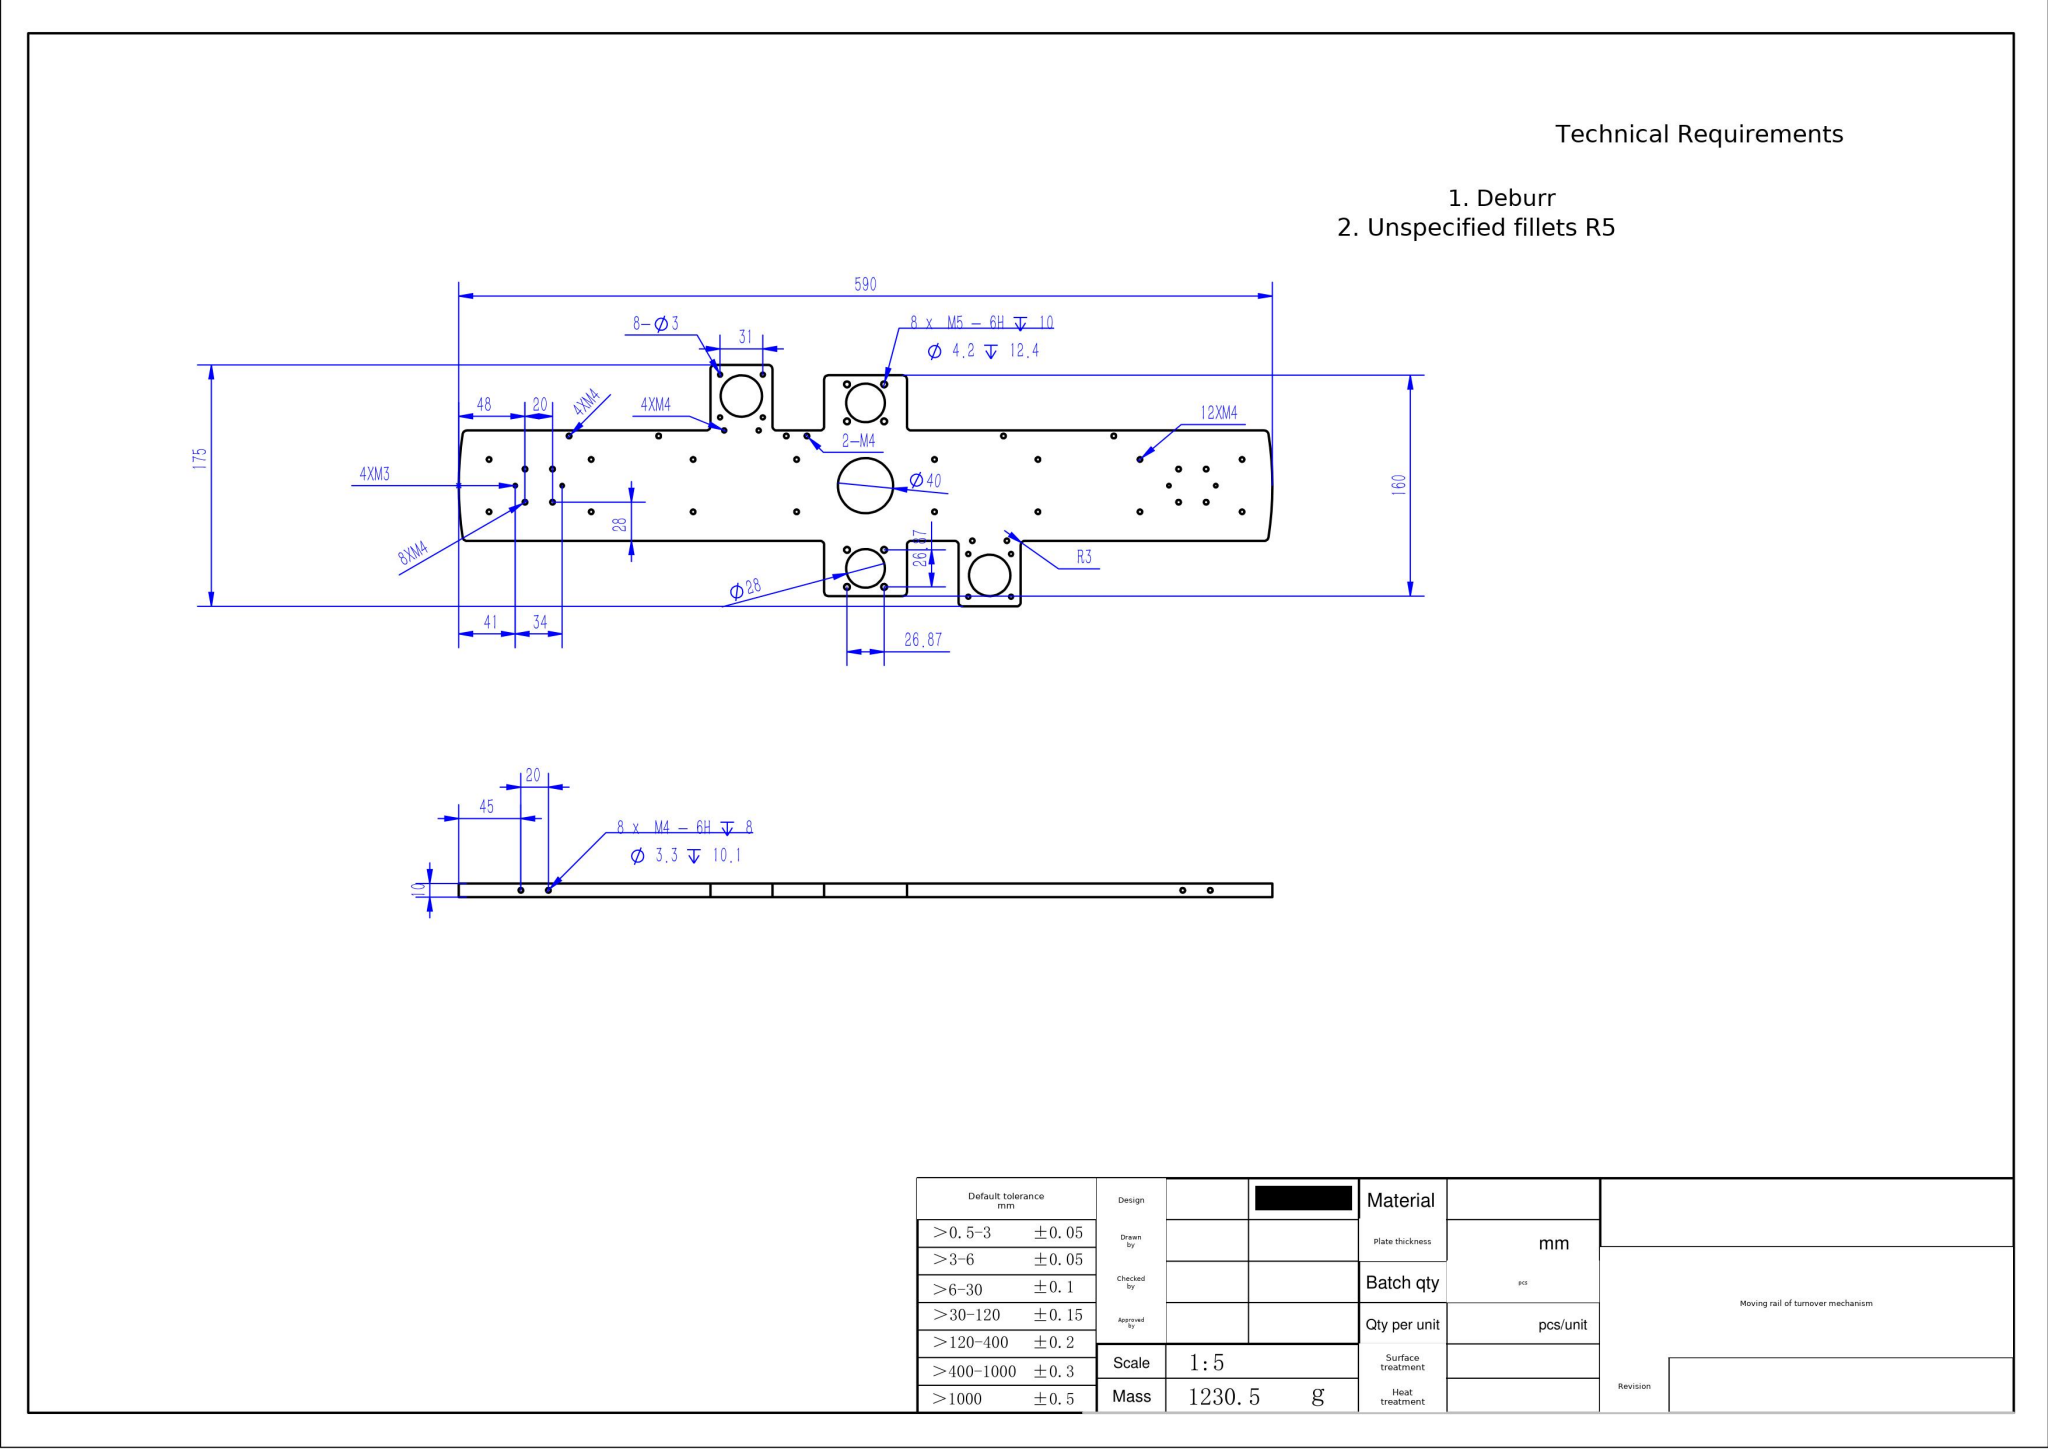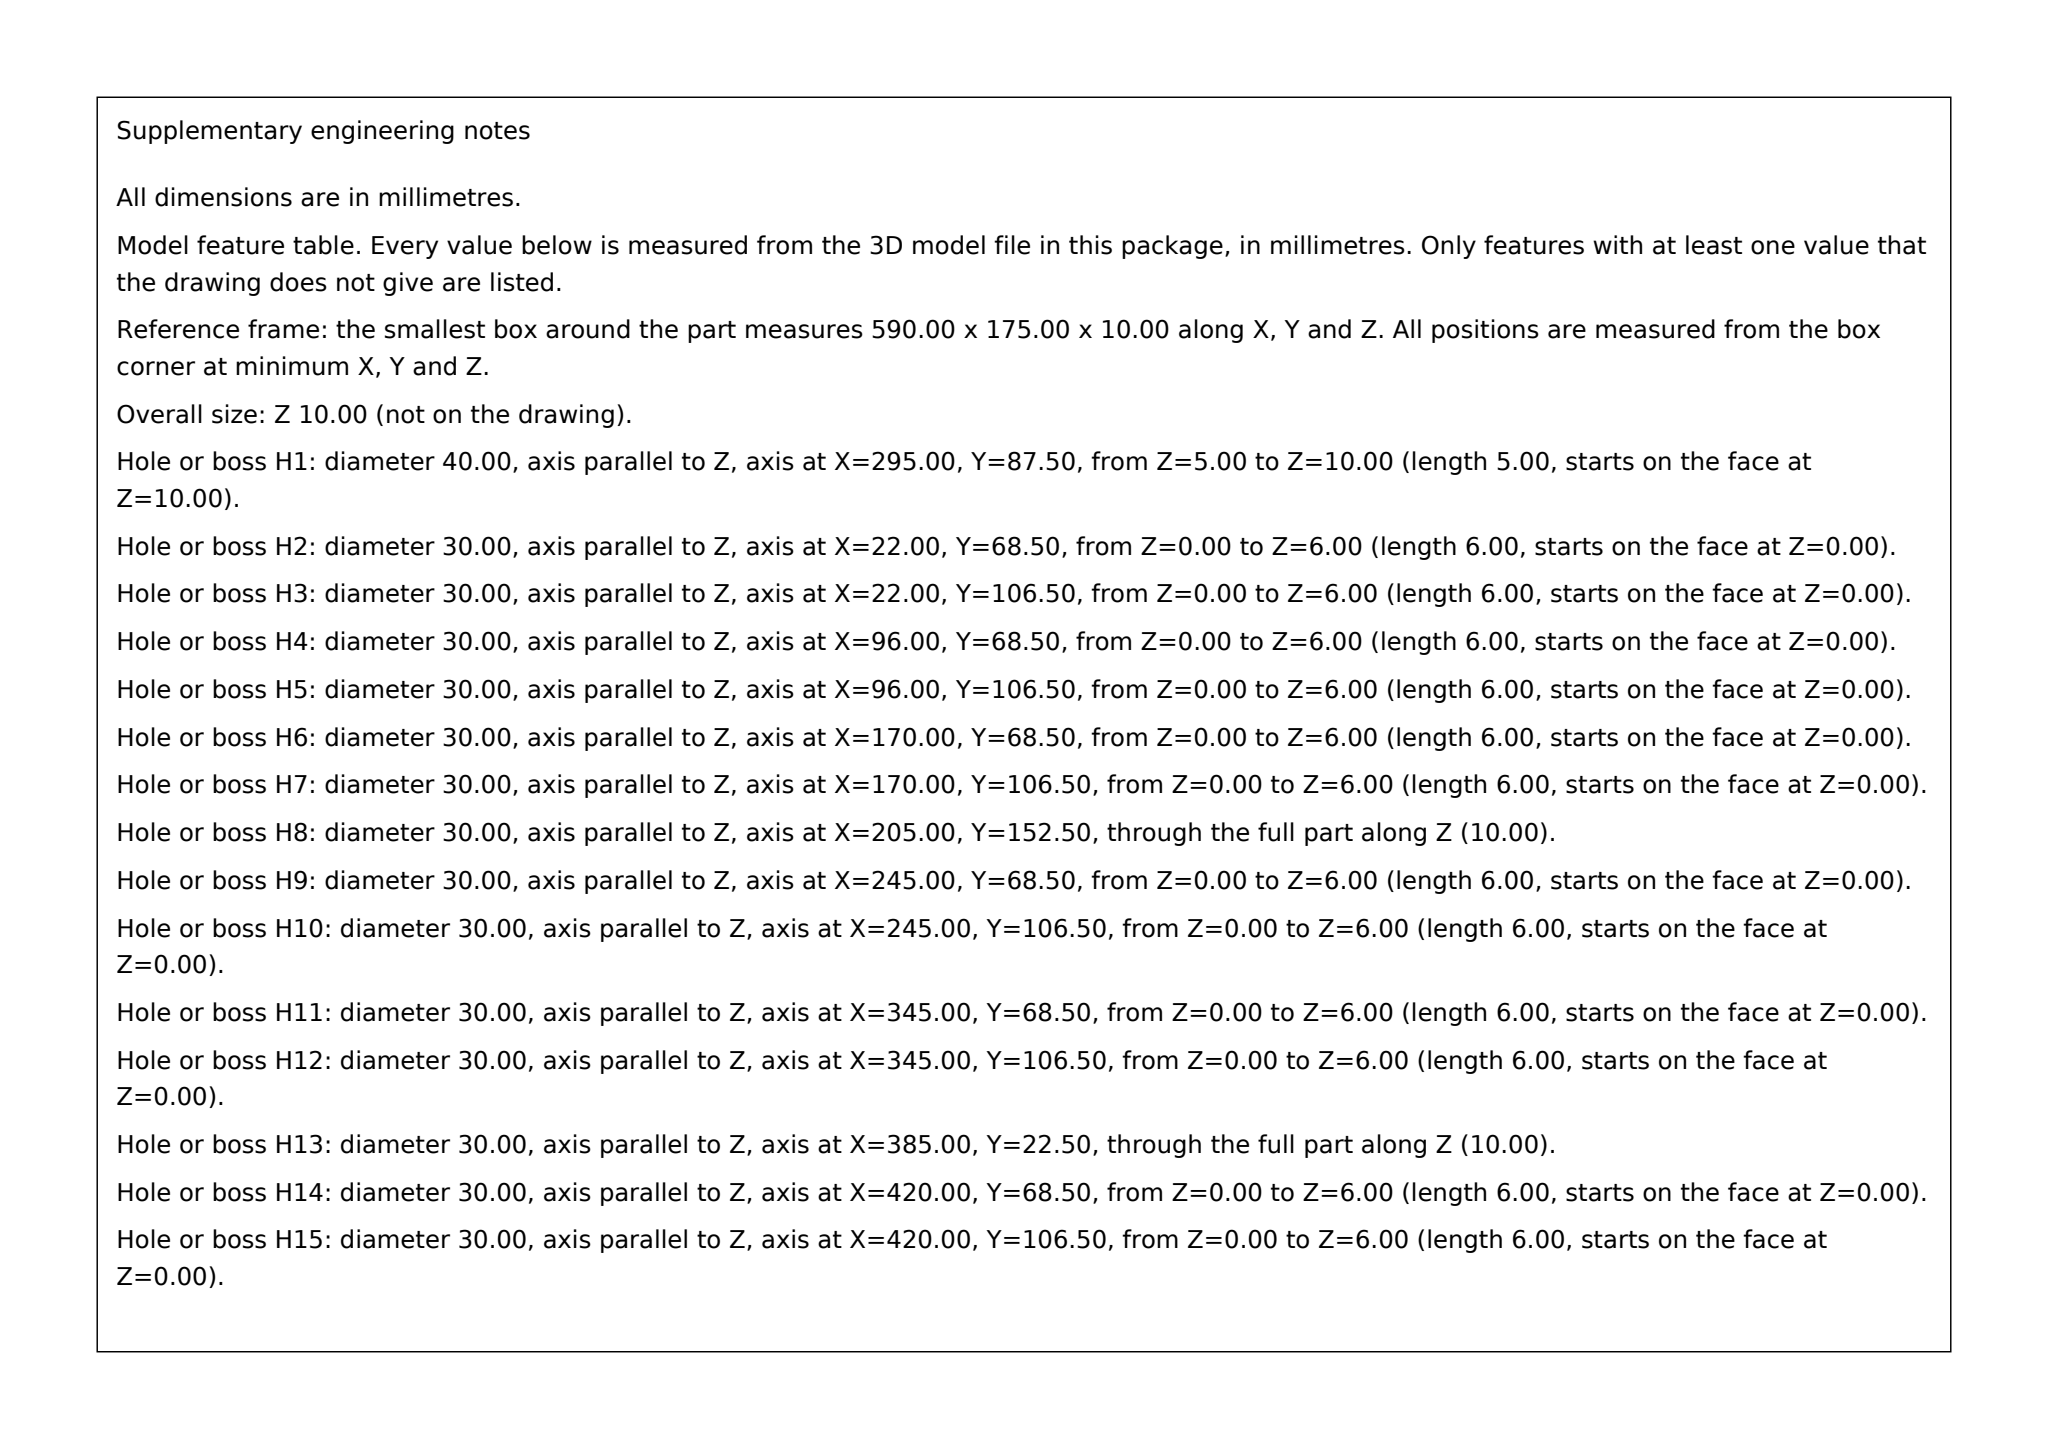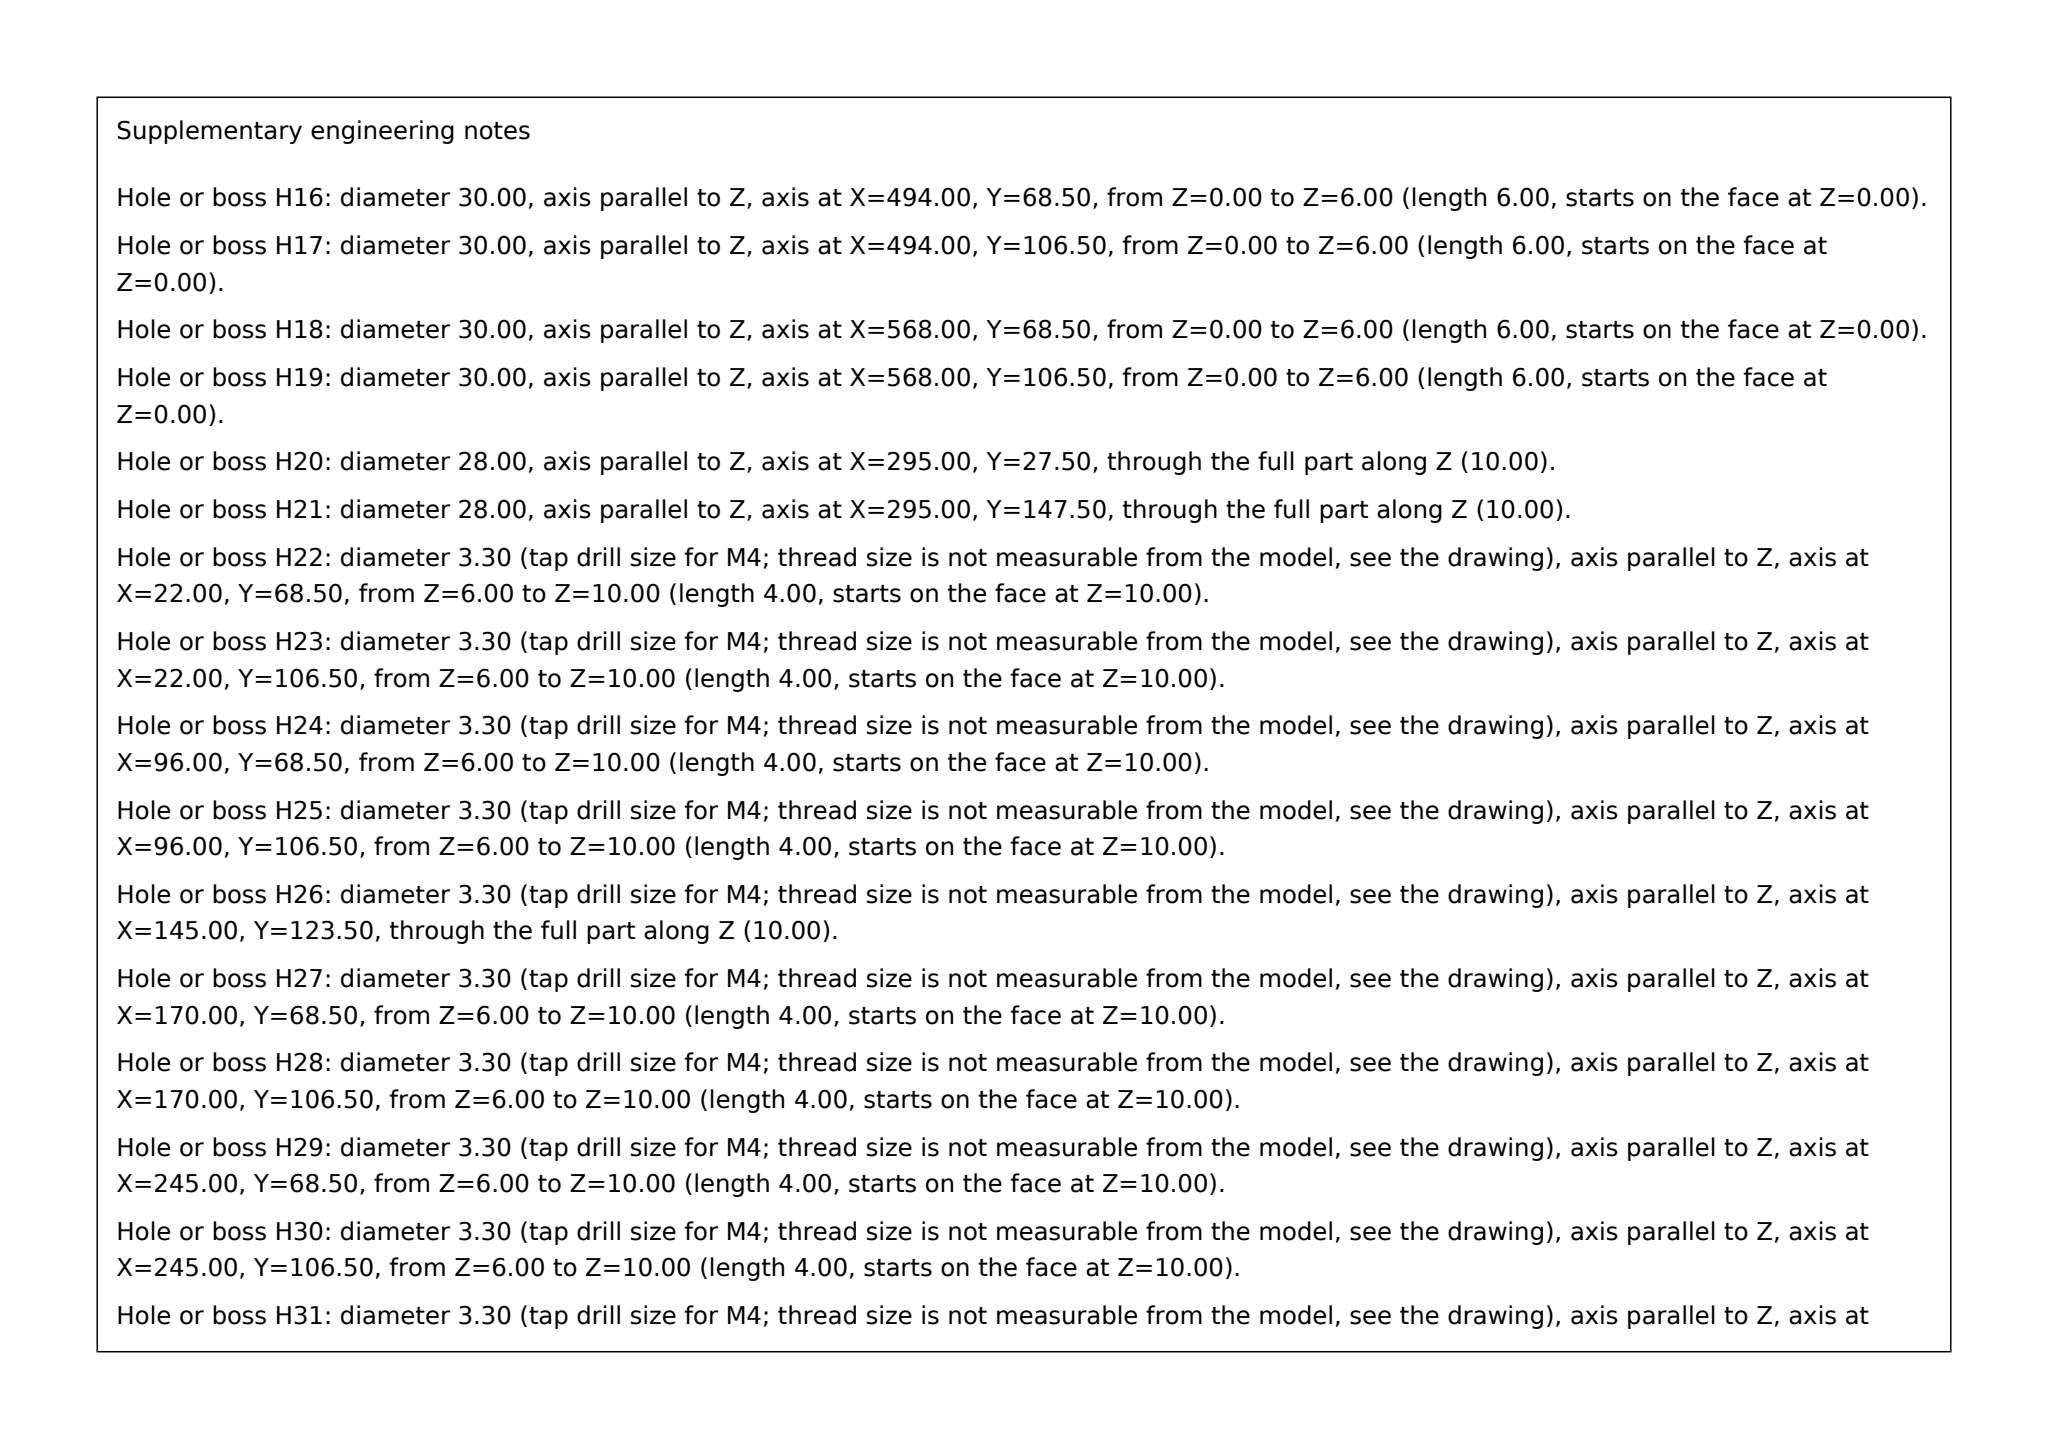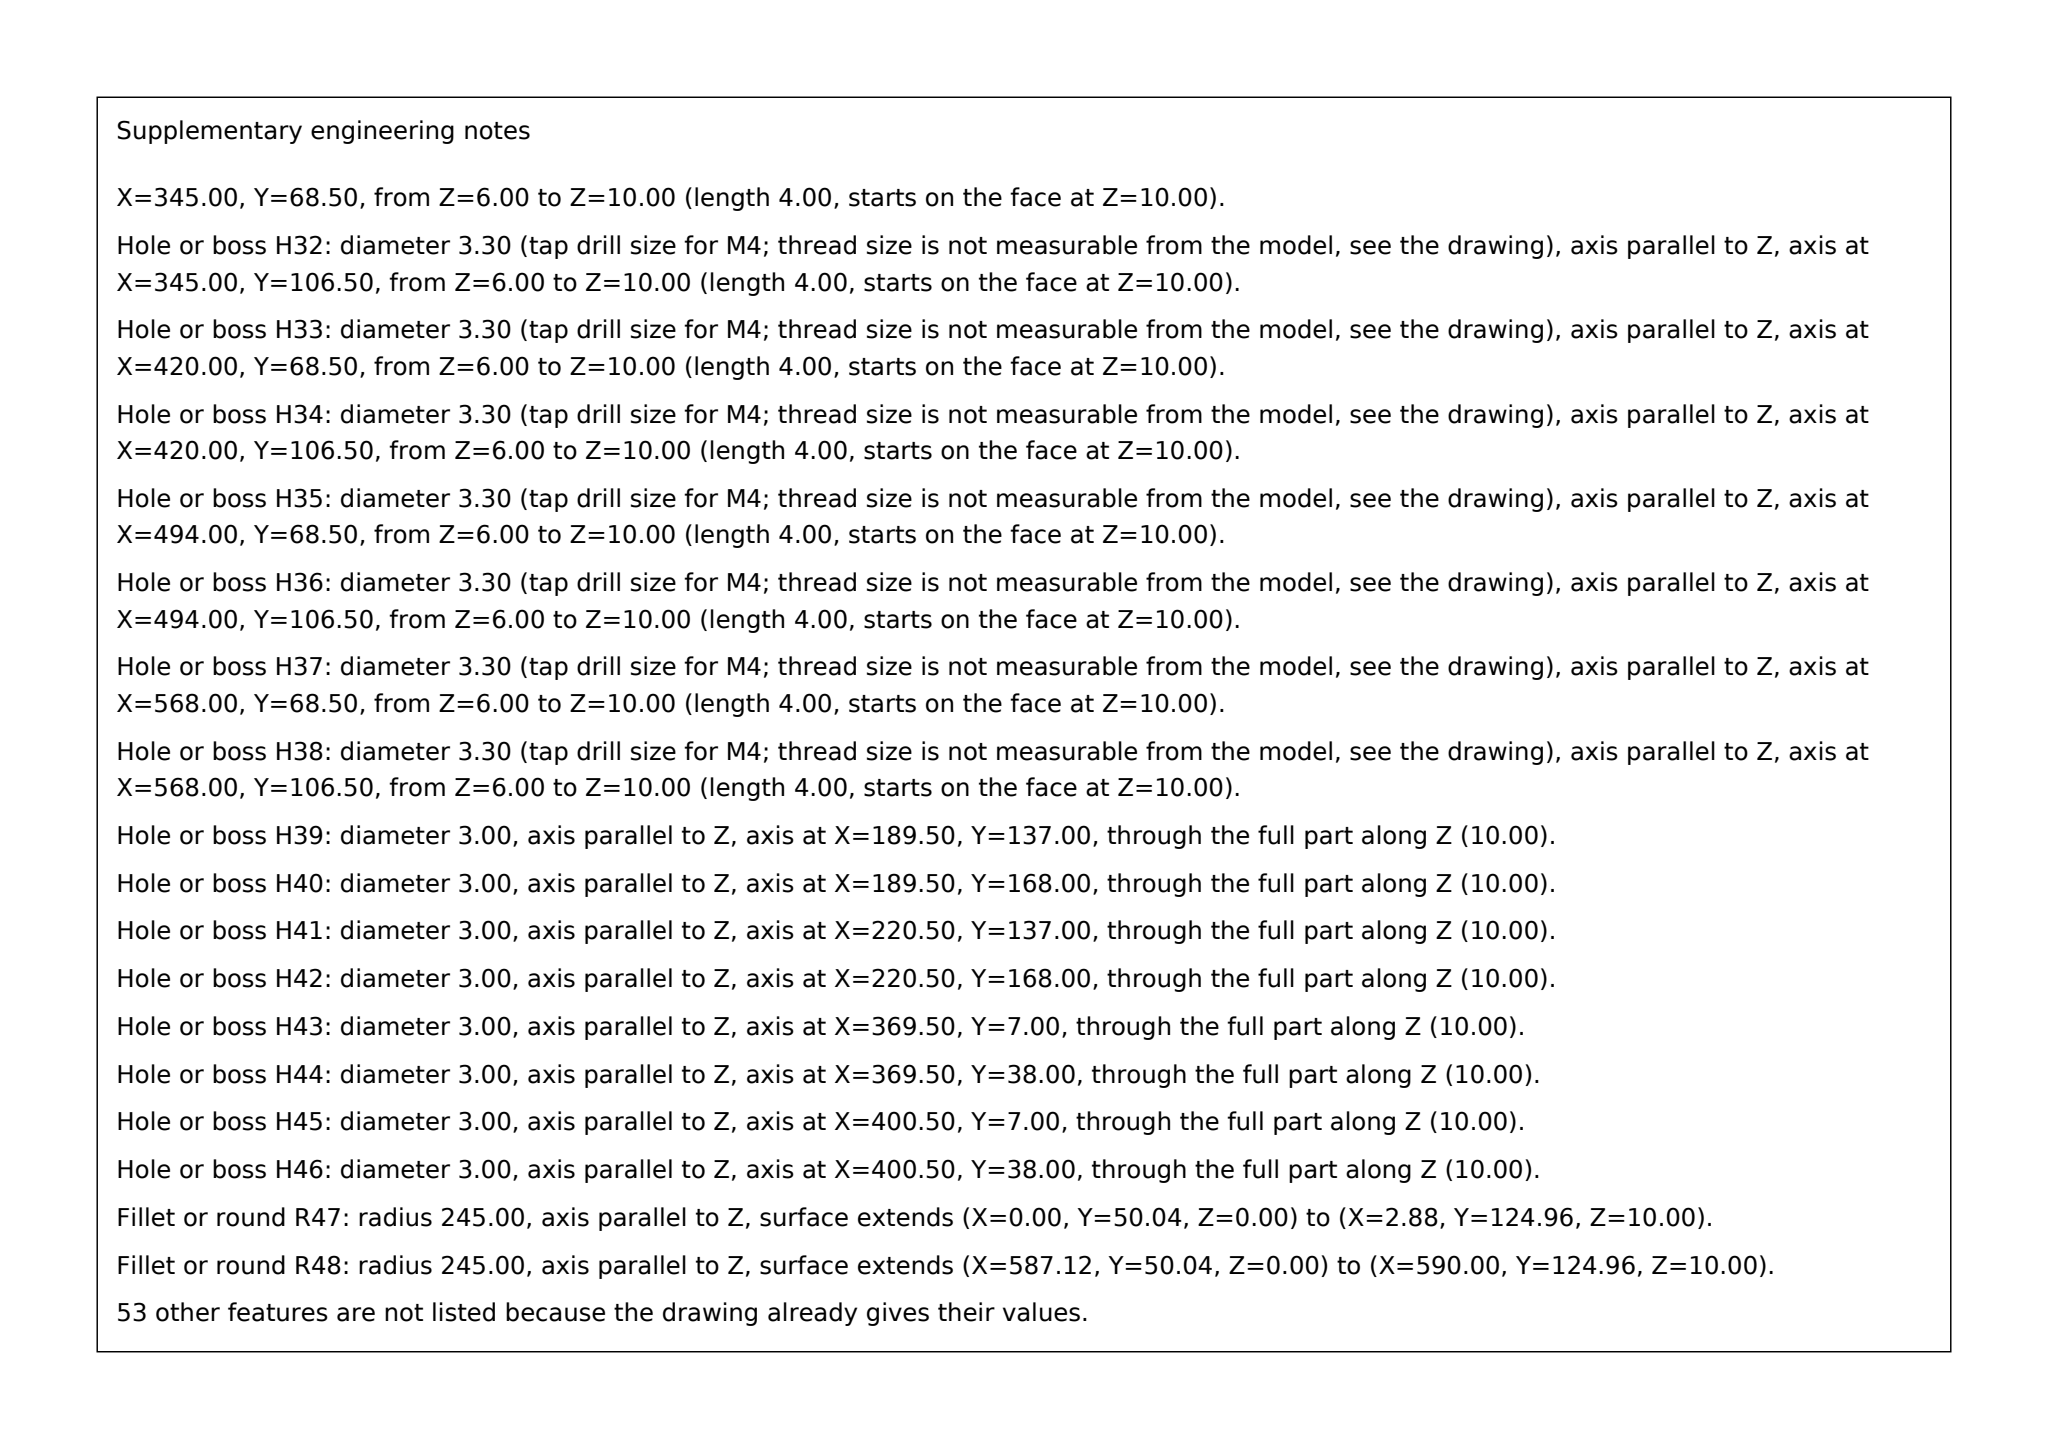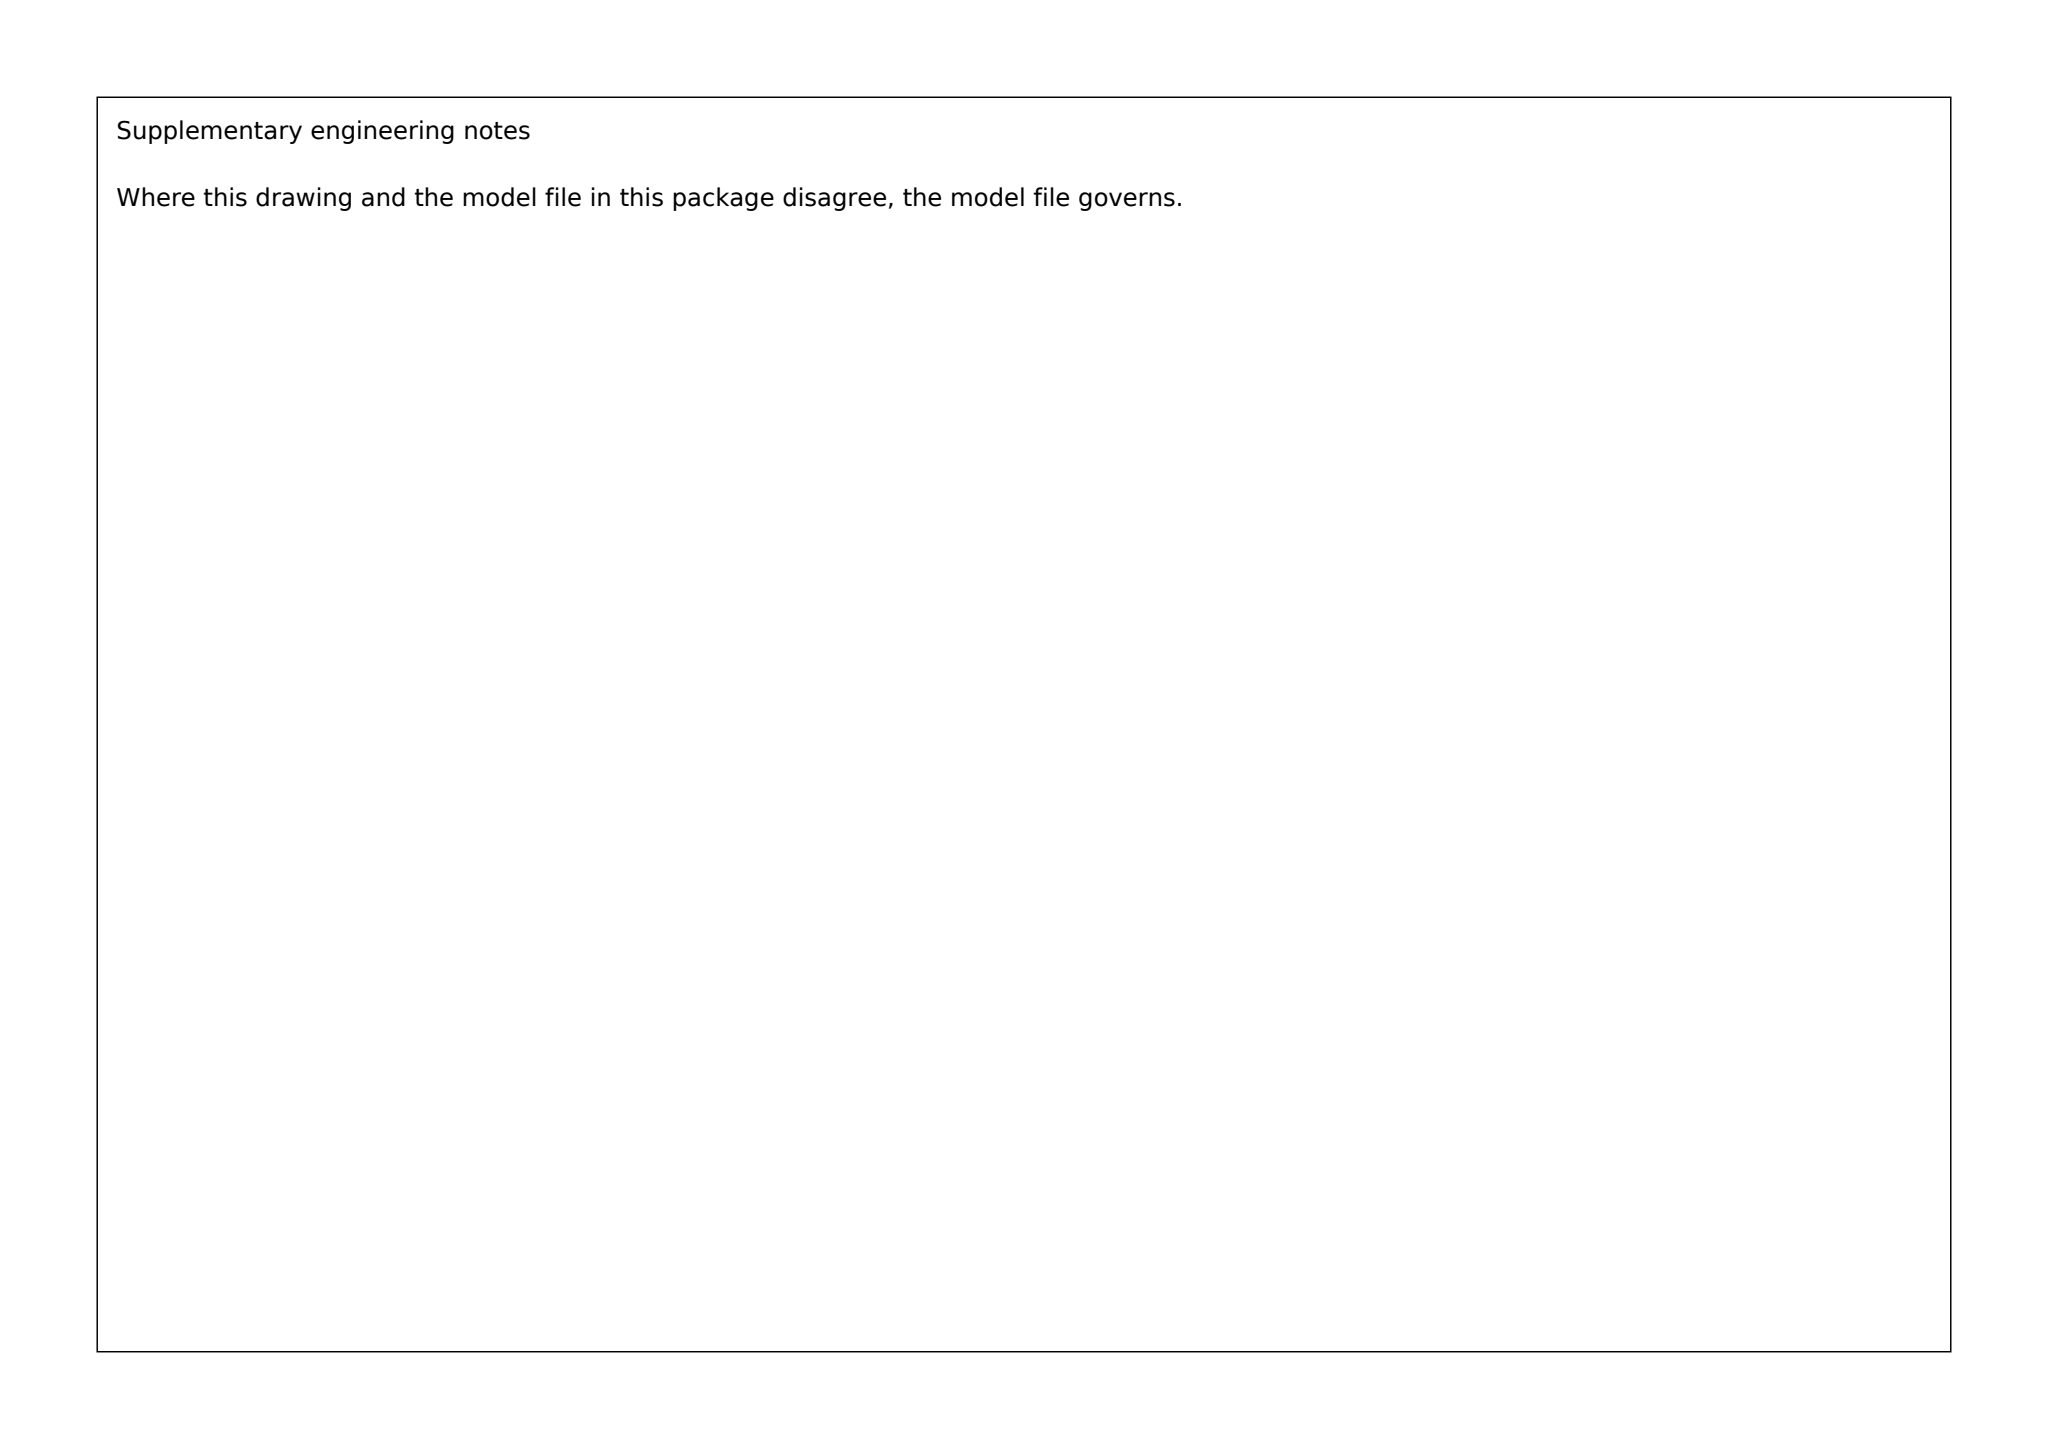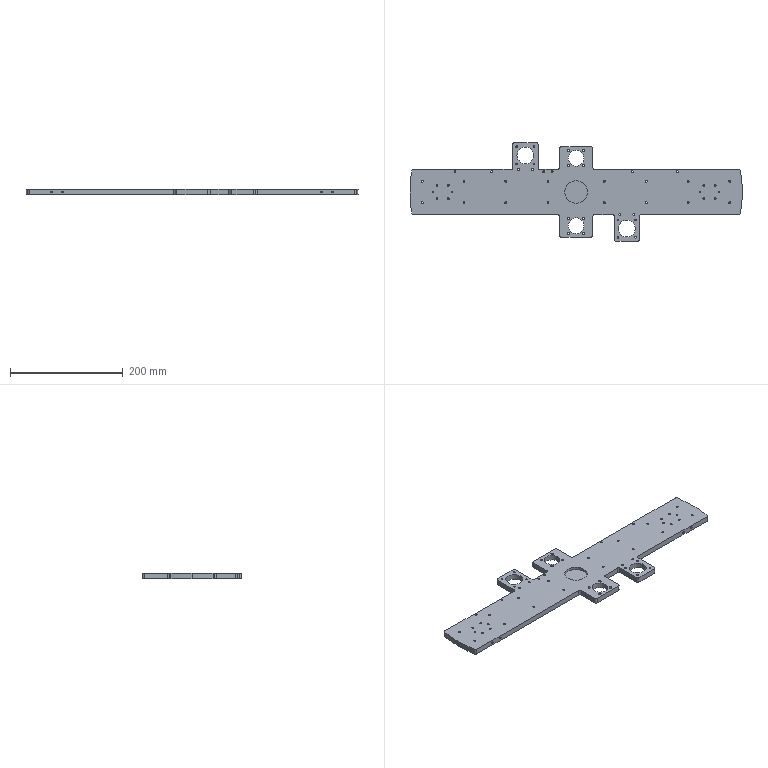Part | SolidWorks | mm | 1 solid | 250 faces | box 590 x 175 x 10 mm | volume 455758 mm3 | cylinder 189 | plane 37 | cone 24 | commonest cylinder face diameters 3.3 x80 30 x36 3 x20 6 x20 4.2 x16 2.5 x8 28 x4 490 x3